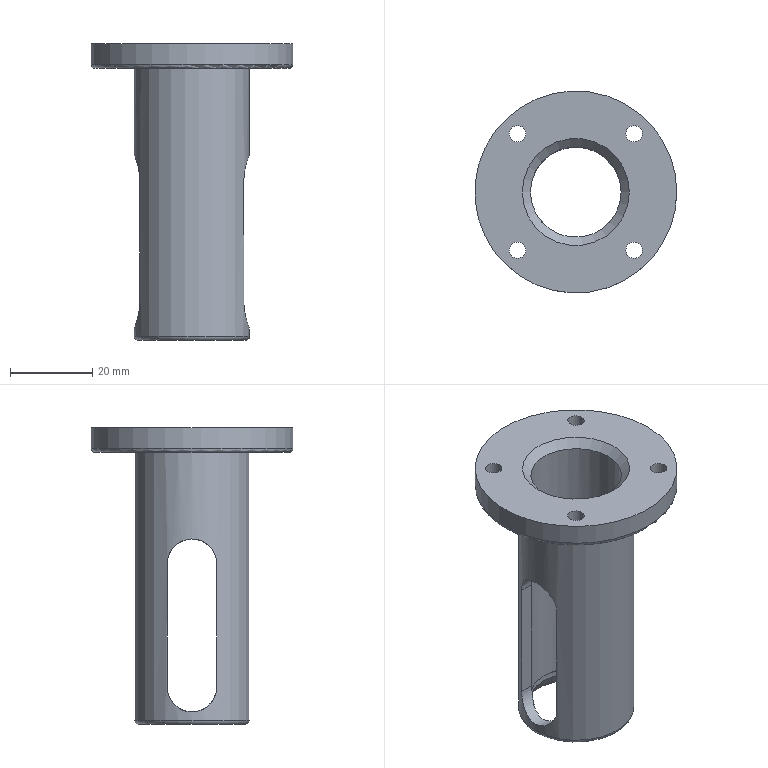Component | NX | 02A__27 | 1 solid | 25 faces | volume 20856 mm3 | cylinder 13 | plane 8 | cone 2 | torus 2 | commonest cylinder face diameters 12 x4 4 x4 22.4 x2 22 x1 28 x1 49 x1